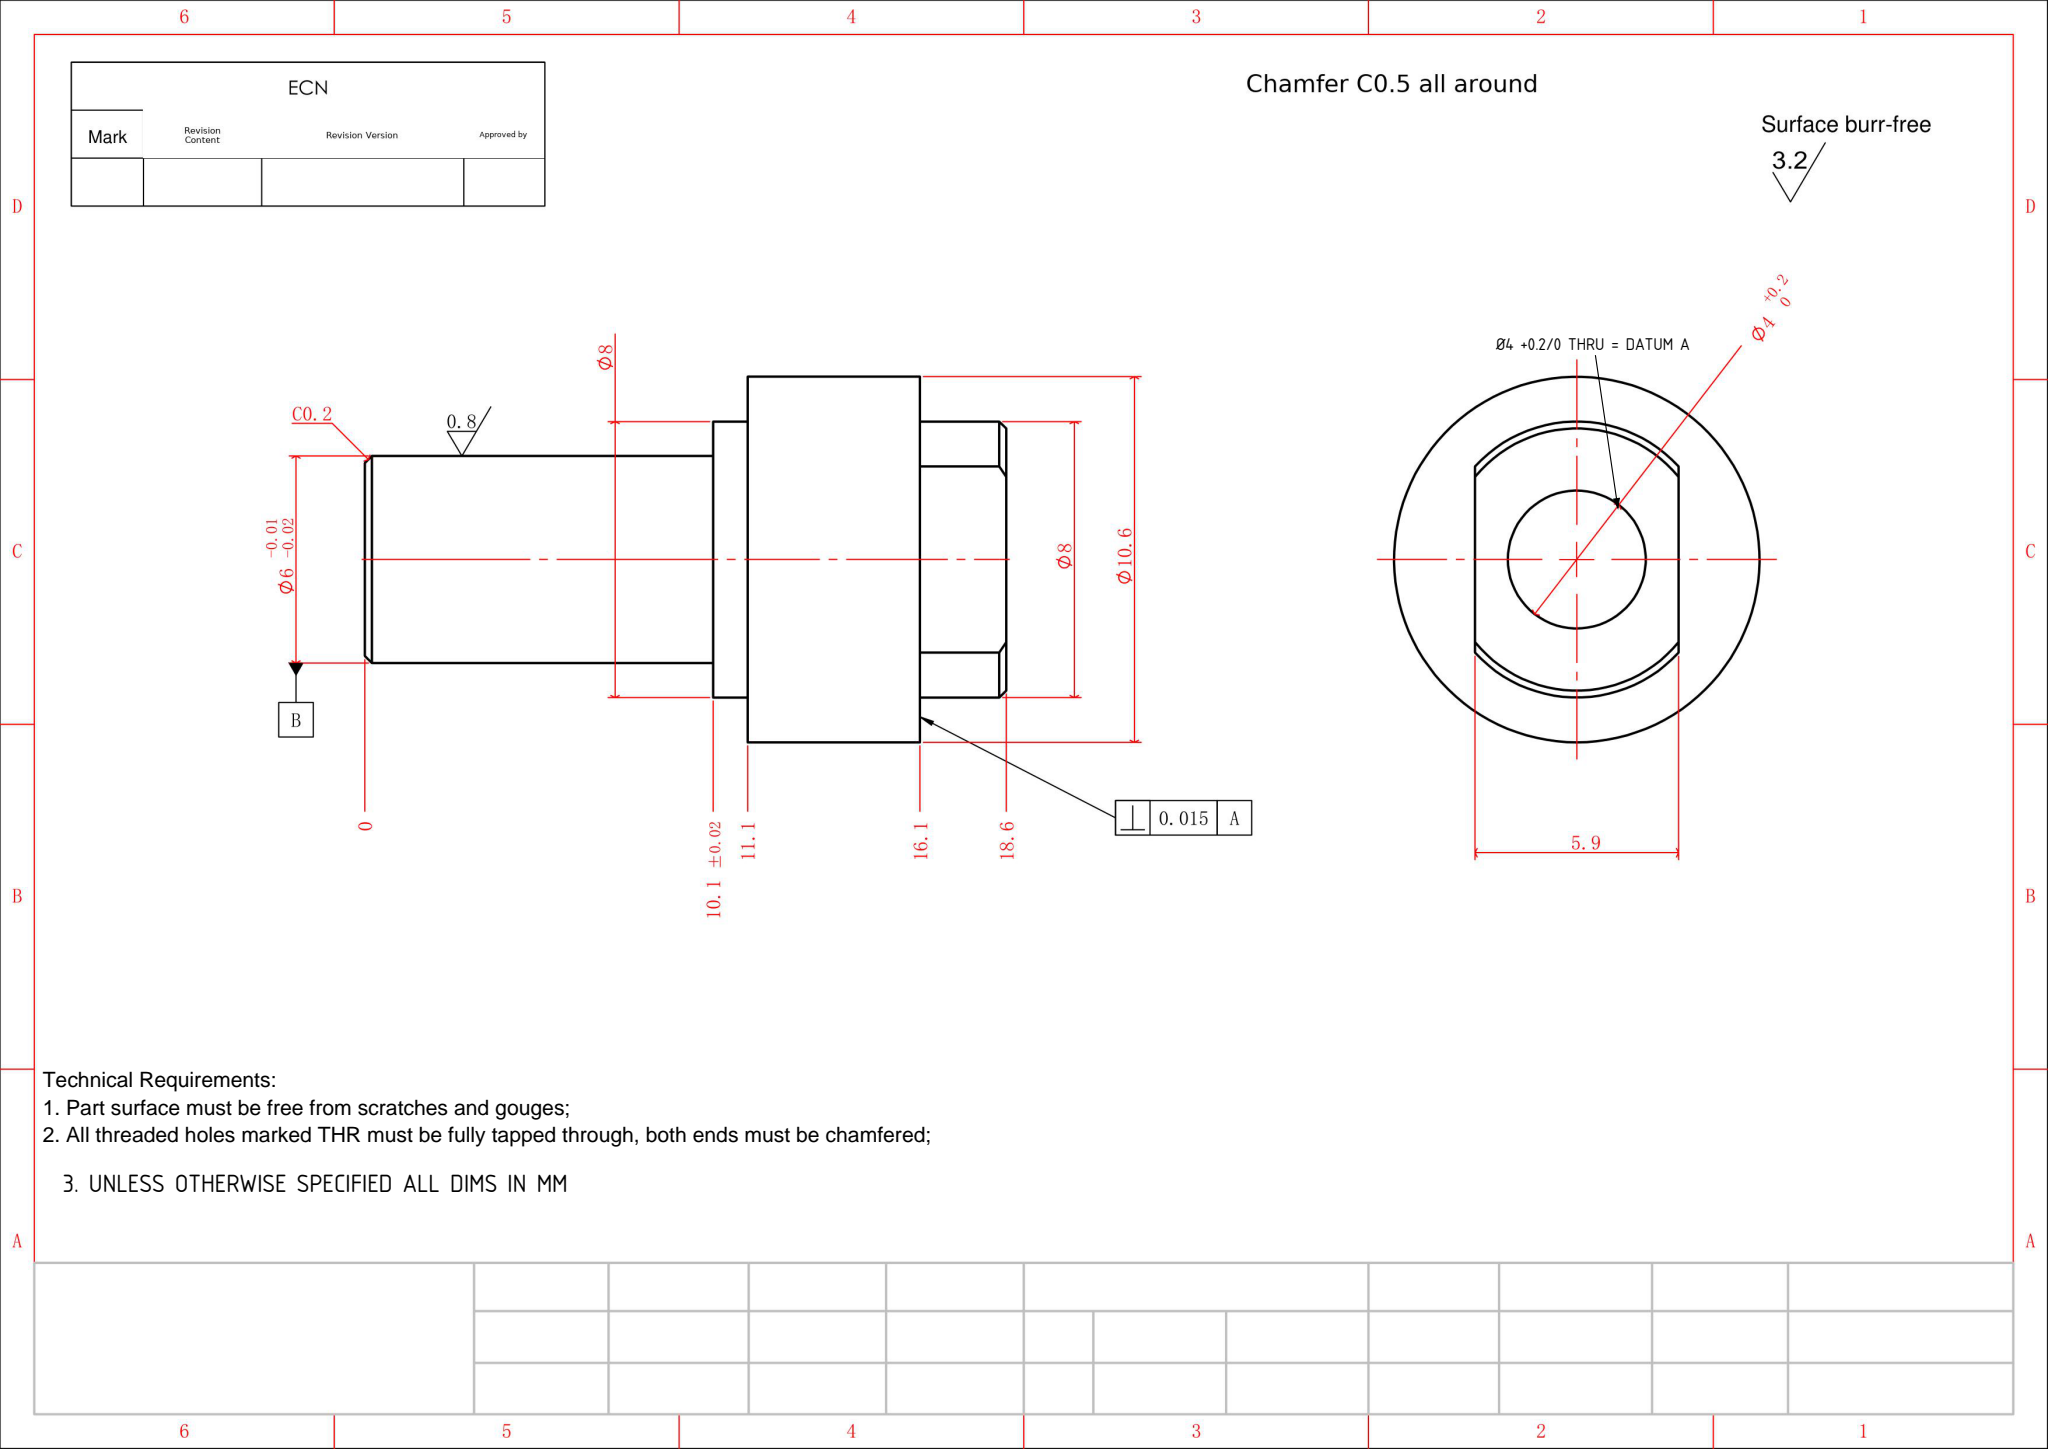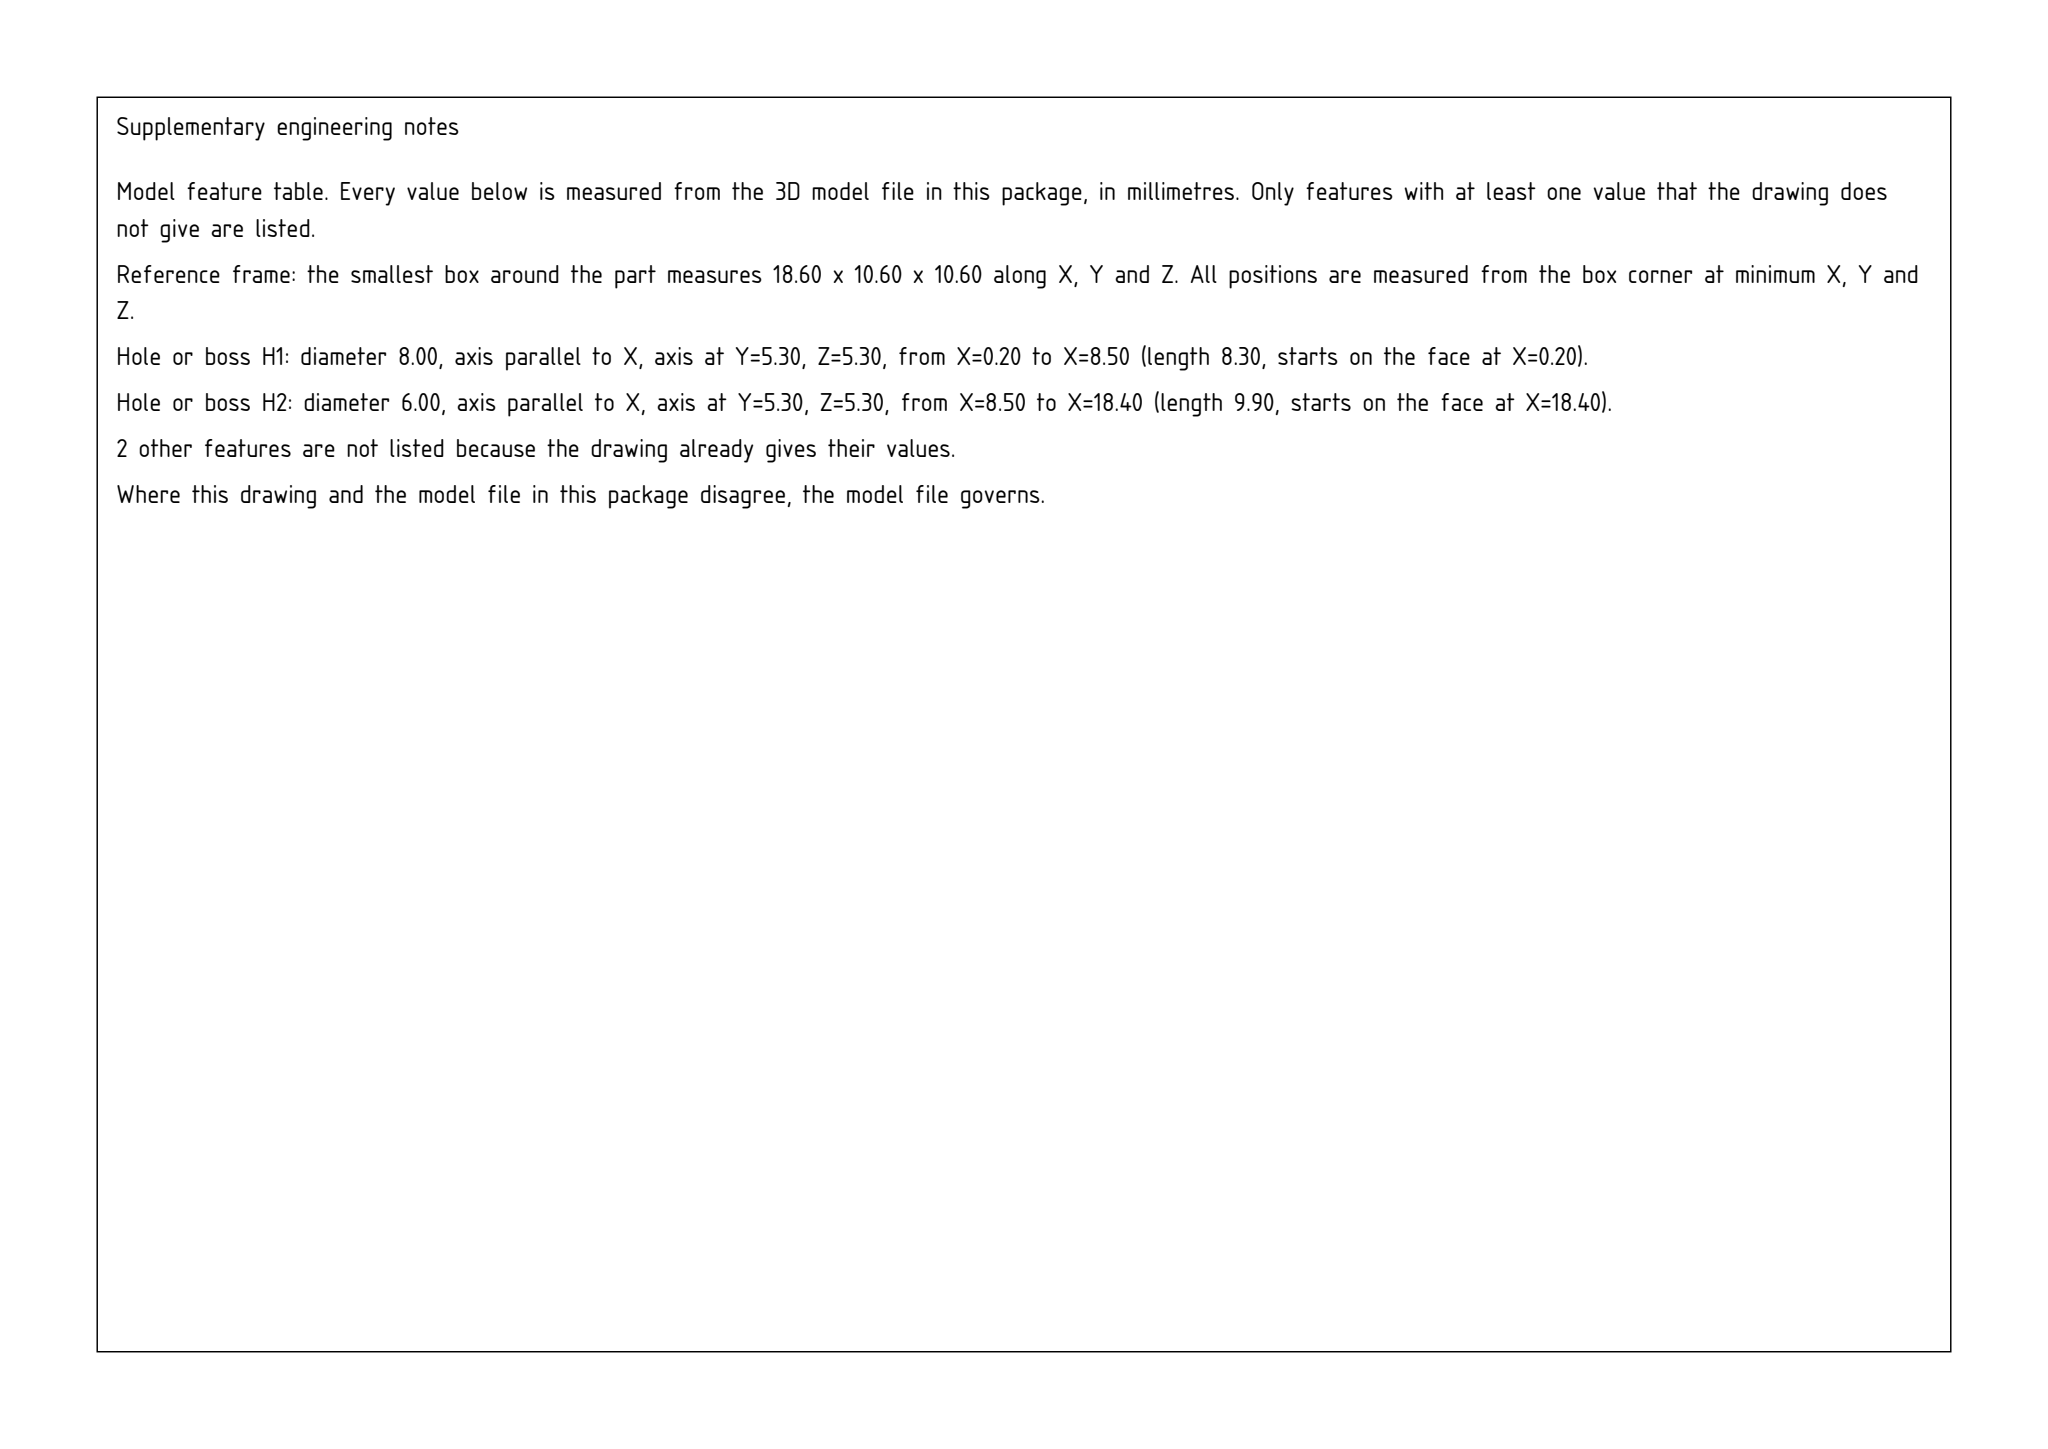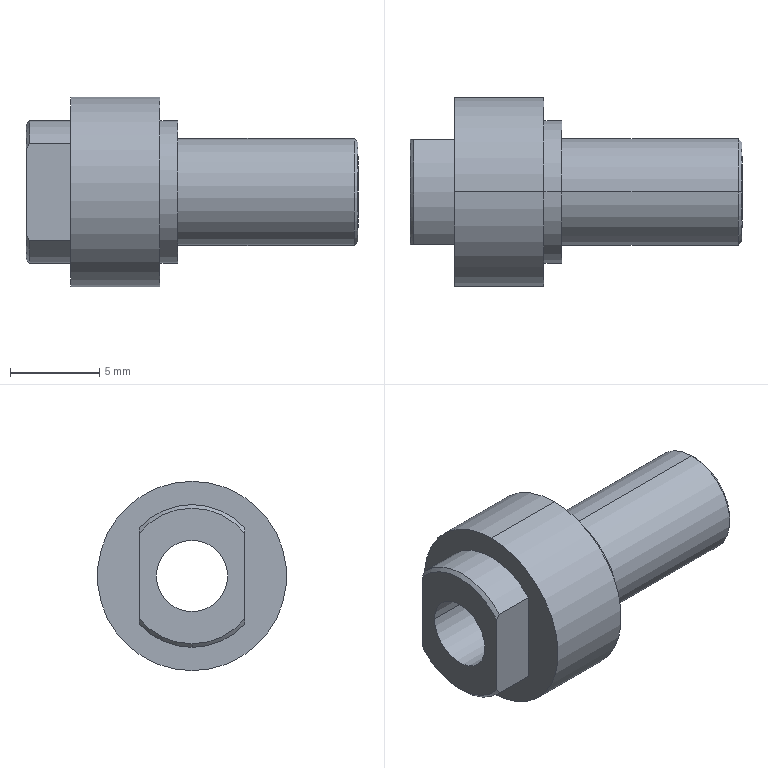Part | SolidWorks | mm | 1 solid | 23 faces | box 18.6 x 10.6 x 10.6 mm | volume 649 mm3 | cylinder 11 | plane 7 | cone 5 | commonest cylinder face diameters 8 x5 4 x2 6 x2 10.6 x2
Drawing notes:
DATUM A = AXIS OF Ø4 +0.2/0 THRU BORE | from the solid: Ø4.0 cylinder, axis x, centered at y=5.3 z=5.3, length 18.6 (full part)
UNLESS OTHERWISE SPECIFIED ALL DIMS IN MM | from the solid: STEP model units mm; bbox 18.6 x 10.6 x 10.6
STEP:
#1=CARTESIAN_POINT('',(-0.,-2.,0.));
#2=VERTEX_POINT('',#1);
#3=CARTESIAN_POINT('',(-0.,2.,0.));
#4=VERTEX_POINT('',#3);
#5=CARTESIAN_POINT('',(-0.,-0.,0.));
#6=DIRECTION('',(1.,0.,0.));
#7=DIRECTION('',(0.,1.,0.));
#8=AXIS2_PLACEMENT_3D('',#5,#6,#7);
#9=CIRCLE('',#8,2.);
#10=EDGE_CURVE('',#2,#4,#9,.T.);
#11=ORIENTED_EDGE('',*,*,#10,.F.);
#12=CARTESIAN_POINT('',(18.6,-2.,0.));
#13=VERTEX_POINT('',#12);
#14=CARTESIAN_POINT('',(-5.289,-2.,0.));
#15=DIRECTION('',(1.,0.,0.));
#16=VECTOR('',#15,1000.);
#17=LINE('',#14,#16);
#18=EDGE_CURVE('',#2,#13,#17,.T.);
#19=ORIENTED_EDGE('',*,*,#18,.T.);
#20=CARTESIAN_POINT('',(18.6,2.,0.));
#21=VERTEX_POINT('',#20);
#22=CARTESIAN_POINT('',(18.6,0.,0.));
#23=DIRECTION('',(-1.,-0.,0.));
#24=DIRECTION('',(0.,1.,0.));
#25=AXIS2_PLACEMENT_3D('',#22,#23,#24);
#26=CIRCLE('',#25,2.);
#27=EDGE_CURVE('',#21,#13,#26,.T.);
#28=ORIENTED_EDGE('',*,*,#27,.F.);
#29=CARTESIAN_POINT('',(-5.289,2.,0.));
#30=DIRECTION('',(1.,0.,0.));
#31=VECTOR('',#30,1000.);
#32=LINE('',#29,#31);
#33=EDGE_CURVE('',#4,#21,#32,.T.);
#34=ORIENTED_EDGE('',*,*,#33,.F.);
#35=EDGE_LOOP('',(#11,#19,#28,#34));
#36=FACE_OUTER_BOUND('',#35,.T.);
#37=CARTESIAN_POINT('',(-5.289,-0.,0.));
#38=DIRECTION('',(1.,0.,0.));
#39=DIRECTION('',(0.,1.,0.));
#40=AXIS2_PLACEMENT_3D('',#37,#38,#39);
#41=CYLINDRICAL_SURFACE('',#40,2.);
#42=ADVANCED_FACE('',(#36),#41,.F.);
#43=CARTESIAN_POINT('',(0.,0.,-3.8));
#44=VERTEX_POINT('',#43);
#45=CARTESIAN_POINT('',(-0.,-2.95,-2.395));
#46=VERTEX_POINT('',#45);
#47=CARTESIAN_POINT('',(0.,0.,0.));
#48=DIRECTION('',(-1.,0.,0.));
#49=DIRECTION('',(0.,0.,-1.));
#50=AXIS2_PLACEMENT_3D('',#47,#48,#49);
#51=CIRCLE('',#50,3.8);
#52=EDGE_CURVE('',#44,#46,#51,.T.);
#53=ORIENTED_EDGE('',*,*,#52,.F.);
#54=CARTESIAN_POINT('',(0.2,0.,-4.));
#55=VERTEX_POINT('',#54);
#56=CARTESIAN_POINT('',(0.2,0.,-4.));
#57=DIRECTION('',(0.7071,0.,-0.7071));
#58=VECTOR('',#57,1000.);
#59=LINE('',#56,#58);
#60=EDGE_CURVE('',#44,#55,#59,.T.);
#61=ORIENTED_EDGE('',*,*,#60,.T.);
#62=CARTESIAN_POINT('',(0.2,-2.95,-2.701));
#63=VERTEX_POINT('',#62);
#64=CARTESIAN_POINT('',(0.2,0.,0.));
#65=DIRECTION('',(-1.,-0.,0.));
#66=DIRECTION('',(-0.,1.,0.));
#67=AXIS2_PLACEMENT_3D('',#64,#65,#66);
#68=CIRCLE('',#67,4.);
#69=EDGE_CURVE('',#55,#63,#68,.T.);
#70=ORIENTED_EDGE('',*,*,#69,.T.);
#71=CARTESIAN_POINT('',(0.2,-2.95,-2.701));
#72=CARTESIAN_POINT('',(0.1318,-2.95,-2.6));
#73=CARTESIAN_POINT('',(0.06499,-2.95,-2.498));
#74=CARTESIAN_POINT('',(-0.,-2.95,-2.395));
#75=B_SPLINE_CURVE_WITH_KNOTS('',3,(#71,#72,#73,#74),.UNSPECIFIED.,.F.,.F.,(4,4),(0.,0.0003656),.UNSPECIFIED.);
#76=EDGE_CURVE('',#63,#46,#75,.T.);
#77=ORIENTED_EDGE('',*,*,#76,.T.);
#78=EDGE_LOOP('',(#53,#61,#70,#77));
#79=FACE_OUTER_BOUND('',#78,.T.);
#80=CARTESIAN_POINT('',(0.2,0.,0.));
#81=DIRECTION('',(1.,0.,0.));
#82=DIRECTION('',(0.,0.,-1.));
#83=AXIS2_PLACEMENT_3D('',#80,#81,#82);
#84=CONICAL_SURFACE('',#83,4.,0.7854);
#85=ADVANCED_FACE('',(#79),#84,.T.);
#86=CARTESIAN_POINT('',(18.6,0.,-2.8));
#87=VERTEX_POINT('',#86);
#88=CARTESIAN_POINT('',(18.6,0.,2.8));
#89=VERTEX_POINT('',#88);
#90=CARTESIAN_POINT('',(18.6,0.,0.));
#91=DIRECTION('',(1.,0.,0.));
#92=DIRECTION('',(0.,0.,1.));
#93=AXIS2_PLACEMENT_3D('',#90,#91,#92);
#94=CIRCLE('',#93,2.8);
#95=EDGE_CURVE('',#87,#89,#94,.T.);
#96=ORIENTED_EDGE('',*,*,#95,.F.);
#97=CARTESIAN_POINT('',(18.4,0.,-3.));
#98=VERTEX_POINT('',#97);
#99=CARTESIAN_POINT('',(18.4,0.,-3.));
#100=DIRECTION('',(-0.7071,0.,-0.7071));
#101=VECTOR('',#100,1000.);
#102=LINE('',#99,#101);
#103=EDGE_CURVE('',#87,#98,#102,.T.);
#104=ORIENTED_EDGE('',*,*,#103,.T.);
#105=CARTESIAN_POINT('',(18.4,0.,3.));
#106=VERTEX_POINT('',#105);
#107=CARTESIAN_POINT('',(18.4,0.,0.));
#108=DIRECTION('',(1.,0.,0.));
#109=DIRECTION('',(0.,-1.,0.));
#110=AXIS2_PLACEMENT_3D('',#107,#108,#109);
#111=CIRCLE('',#110,3.);
#112=EDGE_CURVE('',#98,#106,#111,.T.);
#113=ORIENTED_EDGE('',*,*,#112,.T.);
#114=CARTESIAN_POINT('',(18.4,0.,3.));
#115=DIRECTION('',(-0.7071,0.,0.7071));
#116=VECTOR('',#115,1000.);
#117=LINE('',#114,#116);
#118=EDGE_CURVE('',#89,#106,#117,.T.);
#119=ORIENTED_EDGE('',*,*,#118,.F.);
#120=EDGE_LOOP('',(#96,#104,#113,#119));
#121=FACE_OUTER_BOUND('',#120,.T.);
#122=CARTESIAN_POINT('',(18.4,0.,0.));
#123=DIRECTION('',(-1.,0.,0.));
#124=DIRECTION('',(0.,0.,1.));
#125=AXIS2_PLACEMENT_3D('',#122,#123,#124);
#126=CONICAL_SURFACE('',#125,3.,0.7854);
#127=ADVANCED_FACE('',(#121),#126,.T.);
#128=ORIENTED_EDGE('',*,*,#69,.F.);
#129=CARTESIAN_POINT('',(2.5,0.,-4.));
#130=VERTEX_POINT('',#129);
#131=CARTESIAN_POINT('',(1.25,0.,-4.));
#132=DIRECTION('',(1.,0.,0.));
#133=VECTOR('',#132,1000.);
#134=LINE('',#131,#133);
#135=EDGE_CURVE('',#55,#130,#134,.T.);
#136=ORIENTED_EDGE('',*,*,#135,.T.);
#137=CARTESIAN_POINT('',(2.5,-2.95,-2.701));
#138=VERTEX_POINT('',#137);
#139=CARTESIAN_POINT('',(2.5,0.,0.));
#140=DIRECTION('',(-1.,0.,0.));
#141=DIRECTION('',(0.,0.,-1.));
#142=AXIS2_PLACEMENT_3D('',#139,#140,#141);
#143=CIRCLE('',#142,4.);
#144=EDGE_CURVE('',#130,#138,#143,.T.);
#145=ORIENTED_EDGE('',*,*,#144,.T.);
#146=CARTESIAN_POINT('',(-0.,-2.95,-2.701));
#147=DIRECTION('',(-1.,0.,0.));
#148=VECTOR('',#147,1000.);
#149=LINE('',#146,#148);
#150=EDGE_CURVE('',#138,#63,#149,.T.);
#151=ORIENTED_EDGE('',*,*,#150,.T.);
#152=EDGE_LOOP('',(#128,#136,#145,#151));
#153=FACE_OUTER_BOUND('',#152,.T.);
#154=CARTESIAN_POINT('',(1.25,0.,0.));
#155=DIRECTION('',(1.,0.,0.));
#156=DIRECTION('',(0.,0.,-1.));
#157=AXIS2_PLACEMENT_3D('',#154,#155,#156);
#158=CYLINDRICAL_SURFACE('',#157,4.);
#159=ADVANCED_FACE('',(#153),#158,.T.);
#160=CARTESIAN_POINT('',(8.5,0.,-3.));
#161=VERTEX_POINT('',#160);
#162=CARTESIAN_POINT('',(8.5,0.,3.));
#163=VERTEX_POINT('',#162);
#164=CARTESIAN_POINT('',(8.5,0.,0.));
#165=DIRECTION('',(1.,0.,0.));
#166=DIRECTION('',(0.,0.,-1.));
#167=AXIS2_PLACEMENT_3D('',#164,#165,#166);
#168=CIRCLE('',#167,3.);
#169=EDGE_CURVE('',#161,#163,#168,.T.);
#170=ORIENTED_EDGE('',*,*,#169,.T.);
#171=CARTESIAN_POINT('',(13.55,0.,3.));
#172=DIRECTION('',(1.,0.,0.));
#173=VECTOR('',#172,1000.);
#174=LINE('',#171,#173);
#175=EDGE_CURVE('',#163,#106,#174,.T.);
#176=ORIENTED_EDGE('',*,*,#175,.T.);
#177=ORIENTED_EDGE('',*,*,#112,.F.);
#178=CARTESIAN_POINT('',(13.55,0.,-3.));
#179=DIRECTION('',(1.,0.,0.));
#180=VECTOR('',#179,1000.);
#181=LINE('',#178,#180);
#182=EDGE_CURVE('',#161,#98,#181,.T.);
#183=ORIENTED_EDGE('',*,*,#182,.F.);
#184=EDGE_LOOP('',(#170,#176,#177,#183));
#185=FACE_OUTER_BOUND('',#184,.T.);
#186=CARTESIAN_POINT('',(13.55,0.,0.));
#187=DIRECTION('',(1.,0.,0.));
#188=DIRECTION('',(0.,0.,-1.));
#189=AXIS2_PLACEMENT_3D('',#186,#187,#188);
#190=CYLINDRICAL_SURFACE('',#189,3.);
#191=ADVANCED_FACE('',(#185),#190,.T.);
#192=CARTESIAN_POINT('',(2.5,0.,5.3));
#193=VERTEX_POINT('',#192);
#194=CARTESIAN_POINT('',(2.5,0.,-5.3));
#195=VERTEX_POINT('',#194);
#196=CARTESIAN_POINT('',(2.5,0.,0.));
#197=DIRECTION('',(-1.,0.,0.));
#198=DIRECTION('',(0.,0.,-1.));
#199=AXIS2_PLACEMENT_3D('',#196,#197,#198);
#200=CIRCLE('',#199,5.3);
#201=EDGE_CURVE('',#193,#195,#200,.T.);
#202=ORIENTED_EDGE('',*,*,#201,.F.);
#203=CARTESIAN_POINT('',(7.5,0.,5.3));
#204=VERTEX_POINT('',#203);
#205=CARTESIAN_POINT('',(5.5,0.,5.3));
#206=DIRECTION('',(1.,0.,0.));
#207=VECTOR('',#206,1000.);
#208=LINE('',#205,#207);
#209=EDGE_CURVE('',#193,#204,#208,.T.);
#210=ORIENTED_EDGE('',*,*,#209,.T.);
#211=CARTESIAN_POINT('',(7.5,0.,-5.3));
#212=VERTEX_POINT('',#211);
#213=CARTESIAN_POINT('',(7.5,0.,0.));
#214=DIRECTION('',(-1.,0.,0.));
#215=DIRECTION('',(0.,0.,-1.));
#216=AXIS2_PLACEMENT_3D('',#213,#214,#215);
#217=CIRCLE('',#216,5.3);
#218=EDGE_CURVE('',#204,#212,#217,.T.);
#219=ORIENTED_EDGE('',*,*,#218,.T.);
#220=CARTESIAN_POINT('',(5.5,0.,-5.3));
#221=DIRECTION('',(1.,0.,0.));
#222=VECTOR('',#221,1000.);
#223=LINE('',#220,#222);
#224=EDGE_CURVE('',#195,#212,#223,.T.);
#225=ORIENTED_EDGE('',*,*,#224,.F.);
#226=EDGE_LOOP('',(#202,#210,#219,#225));
#227=FACE_OUTER_BOUND('',#226,.T.);
#228=CARTESIAN_POINT('',(5.5,0.,0.));
#229=DIRECTION('',(1.,0.,0.));
#230=DIRECTION('',(0.,0.,-1.));
#231=AXIS2_PLACEMENT_3D('',#228,#229,#230);
#232=CYLINDRICAL_SURFACE('',#231,5.3);
#233=ADVANCED_FACE('',(#227),#232,.T.);
#234=CARTESIAN_POINT('',(7.5,0.,-4.));
#235=VERTEX_POINT('',#234);
#236=CARTESIAN_POINT('',(7.5,0.,4.));
#237=VERTEX_POINT('',#236);
#238=CARTESIAN_POINT('',(7.5,0.,0.));
#239=DIRECTION('',(1.,0.,0.));
#240=DIRECTION('',(0.,0.,-1.));
#241=AXIS2_PLACEMENT_3D('',#238,#239,#240);
#242=CIRCLE('',#241,4.);
#243=EDGE_CURVE('',#235,#237,#242,.T.);
#244=ORIENTED_EDGE('',*,*,#243,.T.);
#245=CARTESIAN_POINT('',(8.5,0.,4.));
#246=VERTEX_POINT('',#245);
#247=CARTESIAN_POINT('',(8.,0.,4.));
#248=DIRECTION('',(1.,0.,0.));
#249=VECTOR('',#248,1000.);
#250=LINE('',#247,#249);
#251=EDGE_CURVE('',#237,#246,#250,.T.);
#252=ORIENTED_EDGE('',*,*,#251,.T.);
#253=CARTESIAN_POINT('',(8.5,0.,-4.));
#254=VERTEX_POINT('',#253);
#255=CARTESIAN_POINT('',(8.5,0.,0.));
#256=DIRECTION('',(1.,0.,0.));
#257=DIRECTION('',(0.,0.,-1.));
#258=AXIS2_PLACEMENT_3D('',#255,#256,#257);
#259=CIRCLE('',#258,4.);
#260=EDGE_CURVE('',#254,#246,#259,.T.);
#261=ORIENTED_EDGE('',*,*,#260,.F.);
#262=CARTESIAN_POINT('',(8.,0.,-4.));
#263=DIRECTION('',(1.,0.,0.));
#264=VECTOR('',#263,1000.);
#265=LINE('',#262,#264);
#266=EDGE_CURVE('',#235,#254,#265,.T.);
#267=ORIENTED_EDGE('',*,*,#266,.F.);
#268=EDGE_LOOP('',(#244,#252,#261,#267));
#269=FACE_OUTER_BOUND('',#268,.T.);
#270=CARTESIAN_POINT('',(8.,0.,0.));
#271=DIRECTION('',(1.,0.,0.));
#272=DIRECTION('',(0.,0.,-1.));
#273=AXIS2_PLACEMENT_3D('',#270,#271,#272);
#274=CYLINDRICAL_SURFACE('',#273,4.);
#275=ADVANCED_FACE('',(#269),#274,.T.);
#276=ORIENTED_EDGE('',*,*,#18,.F.);
#277=CARTESIAN_POINT('',(-0.,-0.,0.));
#278=DIRECTION('',(1.,0.,0.));
#279=DIRECTION('',(0.,1.,0.));
#280=AXIS2_PLACEMENT_3D('',#277,#278,#279);
#281=CIRCLE('',#280,2.);
#282=EDGE_CURVE('',#4,#2,#281,.T.);
#283=ORIENTED_EDGE('',*,*,#282,.F.);
#284=ORIENTED_EDGE('',*,*,#33,.T.);
#285=CARTESIAN_POINT('',(18.6,0.,0.));
#286=DIRECTION('',(-1.,-0.,0.));
#287=DIRECTION('',(0.,1.,0.));
#288=AXIS2_PLACEMENT_3D('',#285,#286,#287);
#289=CIRCLE('',#288,2.);
#290=EDGE_CURVE('',#13,#21,#289,.T.);
#291=ORIENTED_EDGE('',*,*,#290,.F.);
#292=EDGE_LOOP('',(#276,#283,#284,#291));
#293=FACE_OUTER_BOUND('',#292,.T.);
#294=CARTESIAN_POINT('',(-5.289,-0.,0.));
#295=DIRECTION('',(1.,0.,0.));
#296=DIRECTION('',(0.,1.,0.));
#297=AXIS2_PLACEMENT_3D('',#294,#295,#296);
#298=CYLINDRICAL_SURFACE('',#297,2.);
#299=ADVANCED_FACE('',(#293),#298,.F.);
#300=ORIENTED_EDGE('',*,*,#282,.T.);
#301=ORIENTED_EDGE('',*,*,#10,.T.);
#302=EDGE_LOOP('',(#300,#301));
#303=FACE_BOUND('',#302,.T.);
#304=CARTESIAN_POINT('',(-0.,2.95,-2.395));
#305=VERTEX_POINT('',#304);
#306=CARTESIAN_POINT('',(0.,0.,0.));
#307=DIRECTION('',(-1.,0.,0.));
#308=DIRECTION('',(0.,0.,-1.));
#309=AXIS2_PLACEMENT_3D('',#306,#307,#308);
#310=CIRCLE('',#309,3.8);
#311=EDGE_CURVE('',#305,#44,#310,.T.);
#312=ORIENTED_EDGE('',*,*,#311,.T.);
#313=ORIENTED_EDGE('',*,*,#52,.T.);
#314=CARTESIAN_POINT('',(-0.,-2.95,2.395));
#315=VERTEX_POINT('',#314);
#316=CARTESIAN_POINT('',(-0.,-2.95,0.));
#317=DIRECTION('',(0.,0.,1.));
#318=VECTOR('',#317,1000.);
#319=LINE('',#316,#318);
#320=EDGE_CURVE('',#46,#315,#319,.T.);
#321=ORIENTED_EDGE('',*,*,#320,.T.);
#322=CARTESIAN_POINT('',(-0.,2.95,2.395));
#323=VERTEX_POINT('',#322);
#324=CARTESIAN_POINT('',(0.,0.,0.));
#325=DIRECTION('',(-1.,0.,0.));
#326=DIRECTION('',(0.,0.,-1.));
#327=AXIS2_PLACEMENT_3D('',#324,#325,#326);
#328=CIRCLE('',#327,3.8);
#329=EDGE_CURVE('',#315,#323,#328,.T.);
#330=ORIENTED_EDGE('',*,*,#329,.T.);
#331=CARTESIAN_POINT('',(-0.,2.95,0.));
#332=DIRECTION('',(0.,0.,-1.));
#333=VECTOR('',#332,1000.);
#334=LINE('',#331,#333);
#335=EDGE_CURVE('',#323,#305,#334,.T.);
#336=ORIENTED_EDGE('',*,*,#335,.T.);
#337=EDGE_LOOP('',(#312,#313,#321,#330,#336));
#338=FACE_OUTER_BOUND('',#337,.T.);
#339=CARTESIAN_POINT('',(-0.,2.,0.));
#340=DIRECTION('',(-1.,-0.,0.));
#341=DIRECTION('',(0.,-1.,0.));
#342=AXIS2_PLACEMENT_3D('',#339,#340,#341);
#343=PLANE('',#342);
#344=ADVANCED_FACE('',(#303,#338),#343,.T.);
#345=ORIENTED_EDGE('',*,*,#27,.T.);
#346=ORIENTED_EDGE('',*,*,#290,.T.);
#347=EDGE_LOOP('',(#345,#346));
#348=FACE_BOUND('',#347,.T.);
#349=CARTESIAN_POINT('',(18.6,0.,0.));
#350=DIRECTION('',(1.,0.,0.));
#351=DIRECTION('',(0.,0.,1.));
#352=AXIS2_PLACEMENT_3D('',#349,#350,#351);
#353=CIRCLE('',#352,2.8);
#354=EDGE_CURVE('',#89,#87,#353,.T.);
#355=ORIENTED_EDGE('',*,*,#354,.T.);
#356=ORIENTED_EDGE('',*,*,#95,.T.);
#357=EDGE_LOOP('',(#355,#356));
#358=FACE_OUTER_BOUND('',#357,.T.);
#359=CARTESIAN_POINT('',(18.6,1.5,0.));
#360=DIRECTION('',(1.,0.,0.));
#361=DIRECTION('',(0.,0.,-1.));
#362=AXIS2_PLACEMENT_3D('',#359,#360,#361);
#363=PLANE('',#362);
#364=ADVANCED_FACE('',(#348,#358),#363,.T.);
#365=ORIENTED_EDGE('',*,*,#320,.F.);
#366=ORIENTED_EDGE('',*,*,#76,.F.);
#367=ORIENTED_EDGE('',*,*,#150,.F.);
#368=CARTESIAN_POINT('',(2.5,-2.95,2.701));
#369=VERTEX_POINT('',#368);
#370=CARTESIAN_POINT('',(2.5,-2.95,2.701));
#371=DIRECTION('',(0.,0.,-1.));
#372=VECTOR('',#371,1000.);
#373=LINE('',#370,#372);
#374=EDGE_CURVE('',#369,#138,#373,.T.);
#375=ORIENTED_EDGE('',*,*,#374,.F.);
#376=CARTESIAN_POINT('',(0.2,-2.95,2.701));
#377=VERTEX_POINT('',#376);
#378=CARTESIAN_POINT('',(-0.,-2.95,2.701));
#379=DIRECTION('',(1.,0.,0.));
#380=VECTOR('',#379,1000.);
#381=LINE('',#378,#380);
#382=EDGE_CURVE('',#377,#369,#381,.T.);
#383=ORIENTED_EDGE('',*,*,#382,.F.);
#384=CARTESIAN_POINT('',(-0.,-2.95,2.395));
#385=CARTESIAN_POINT('',(0.06499,-2.95,2.498));
#386=CARTESIAN_POINT('',(0.1318,-2.95,2.6));
#387=CARTESIAN_POINT('',(0.2,-2.95,2.701));
#388=B_SPLINE_CURVE_WITH_KNOTS('',3,(#384,#385,#386,#387),.UNSPECIFIED.,.F.,.F.,(4,4),(0.,0.0003656),.UNSPECIFIED.);
#389=EDGE_CURVE('',#315,#377,#388,.T.);
#390=ORIENTED_EDGE('',*,*,#389,.F.);
#391=EDGE_LOOP('',(#365,#366,#367,#375,#383,#390));
#392=FACE_OUTER_BOUND('',#391,.T.);
#393=CARTESIAN_POINT('',(-0.,-2.95,2.701));
#394=DIRECTION('',(0.,1.,0.));
#395=DIRECTION('',(0.,0.,1.));
#396=AXIS2_PLACEMENT_3D('',#393,#394,#395);
#397=PLANE('',#396);
#398=ADVANCED_FACE('',(#392),#397,.F.);
#399=ORIENTED_EDGE('',*,*,#60,.F.);
#400=ORIENTED_EDGE('',*,*,#311,.F.);
#401=CARTESIAN_POINT('',(0.2,2.95,-2.701));
#402=VERTEX_POINT('',#401);
#403=CARTESIAN_POINT('',(-0.,2.95,-2.395));
#404=CARTESIAN_POINT('',(0.06499,2.95,-2.498));
#405=CARTESIAN_POINT('',(0.1318,2.95,-2.6));
#406=CARTESIAN_POINT('',(0.2,2.95,-2.701));
#407=B_SPLINE_CURVE_WITH_KNOTS('',3,(#403,#404,#405,#406),.UNSPECIFIED.,.F.,.F.,(4,4),(0.,0.0003656),.UNSPECIFIED.);
#408=EDGE_CURVE('',#305,#402,#407,.T.);
#409=ORIENTED_EDGE('',*,*,#408,.T.);
#410=CARTESIAN_POINT('',(0.2,0.,0.));
#411=DIRECTION('',(-1.,-0.,0.));
#412=DIRECTION('',(-0.,1.,0.));
#413=AXIS2_PLACEMENT_3D('',#410,#411,#412);
#414=CIRCLE('',#413,4.);
#415=EDGE_CURVE('',#402,#55,#414,.T.);
#416=ORIENTED_EDGE('',*,*,#415,.T.);
#417=EDGE_LOOP('',(#399,#400,#409,#416));
#418=FACE_OUTER_BOUND('',#417,.T.);
#419=CARTESIAN_POINT('',(0.2,0.,0.));
#420=DIRECTION('',(1.,0.,0.));
#421=DIRECTION('',(0.,0.,-1.));
#422=AXIS2_PLACEMENT_3D('',#419,#420,#421);
#423=CONICAL_SURFACE('',#422,4.,0.7854);
#424=ADVANCED_FACE('',(#418),#423,.T.);
#425=CARTESIAN_POINT('',(2.5,2.95,2.701));
#426=VERTEX_POINT('',#425);
#427=CARTESIAN_POINT('',(0.2,2.95,2.701));
#428=VERTEX_POINT('',#427);
#429=CARTESIAN_POINT('',(-0.,2.95,2.701));
#430=DIRECTION('',(-1.,0.,0.));
#431=VECTOR('',#430,1000.);
#432=LINE('',#429,#431);
#433=EDGE_CURVE('',#426,#428,#432,.T.);
#434=ORIENTED_EDGE('',*,*,#433,.F.);
#435=CARTESIAN_POINT('',(2.5,2.95,-2.701));
#436=VERTEX_POINT('',#435);
#437=CARTESIAN_POINT('',(2.5,2.95,-2.701));
#438=DIRECTION('',(0.,0.,1.));
#439=VECTOR('',#438,1000.);
#440=LINE('',#437,#439);
#441=EDGE_CURVE('',#436,#426,#440,.T.);
#442=ORIENTED_EDGE('',*,*,#441,.F.);
#443=CARTESIAN_POINT('',(-0.,2.95,-2.701));
#444=DIRECTION('',(1.,0.,0.));
#445=VECTOR('',#444,1000.);
#446=LINE('',#443,#445);
#447=EDGE_CURVE('',#402,#436,#446,.T.);
#448=ORIENTED_EDGE('',*,*,#447,.F.);
#449=ORIENTED_EDGE('',*,*,#408,.F.);
#450=ORIENTED_EDGE('',*,*,#335,.F.);
#451=CARTESIAN_POINT('',(0.2,2.95,2.701));
#452=CARTESIAN_POINT('',(0.1318,2.95,2.6));
#453=CARTESIAN_POINT('',(0.06499,2.95,2.498));
#454=CARTESIAN_POINT('',(-0.,2.95,2.395));
#455=B_SPLINE_CURVE_WITH_KNOTS('',3,(#451,#452,#453,#454),.UNSPECIFIED.,.F.,.F.,(4,4),(0.,0.0003656),.UNSPECIFIED.);
#456=EDGE_CURVE('',#428,#323,#455,.T.);
#457=ORIENTED_EDGE('',*,*,#456,.F.);
#458=EDGE_LOOP('',(#434,#442,#448,#449,#450,#457));
#459=FACE_OUTER_BOUND('',#458,.T.);
#460=CARTESIAN_POINT('',(-0.,2.95,-2.701));
#461=DIRECTION('',(0.,-1.,0.));
#462=DIRECTION('',(0.,0.,-1.));
#463=AXIS2_PLACEMENT_3D('',#460,#461,#462);
#464=PLANE('',#463);
#465=ADVANCED_FACE('',(#459),#464,.F.);
#466=ORIENTED_EDGE('',*,*,#456,.T.);
#467=ORIENTED_EDGE('',*,*,#329,.F.);
#468=ORIENTED_EDGE('',*,*,#389,.T.);
#469=CARTESIAN_POINT('',(0.2,0.,0.));
#470=DIRECTION('',(-1.,-0.,0.));
#471=DIRECTION('',(-0.,1.,0.));
#472=AXIS2_PLACEMENT_3D('',#469,#470,#471);
#473=CIRCLE('',#472,4.);
#474=EDGE_CURVE('',#377,#428,#473,.T.);
#475=ORIENTED_EDGE('',*,*,#474,.T.);
#476=EDGE_LOOP('',(#466,#467,#468,#475));
#477=FACE_OUTER_BOUND('',#476,.T.);
#478=CARTESIAN_POINT('',(0.2,0.,0.));
#479=DIRECTION('',(1.,0.,0.));
#480=DIRECTION('',(0.,0.,-1.));
#481=AXIS2_PLACEMENT_3D('',#478,#479,#480);
#482=CONICAL_SURFACE('',#481,4.,0.7854);
#483=ADVANCED_FACE('',(#477),#482,.T.);
#484=ORIENTED_EDGE('',*,*,#103,.F.);
#485=ORIENTED_EDGE('',*,*,#354,.F.);
#486=ORIENTED_EDGE('',*,*,#118,.T.);
#487=CARTESIAN_POINT('',(18.4,0.,0.));
#488=DIRECTION('',(1.,0.,0.));
#489=DIRECTION('',(0.,-1.,0.));
#490=AXIS2_PLACEMENT_3D('',#487,#488,#489);
#491=CIRCLE('',#490,3.);
#492=EDGE_CURVE('',#106,#98,#491,.T.);
#493=ORIENTED_EDGE('',*,*,#492,.T.);
#494=EDGE_LOOP('',(#484,#485,#486,#493));
#495=FACE_OUTER_BOUND('',#494,.T.);
#496=CARTESIAN_POINT('',(18.4,0.,0.));
#497=DIRECTION('',(-1.,0.,0.));
#498=DIRECTION('',(0.,0.,1.));
#499=AXIS2_PLACEMENT_3D('',#496,#497,#498);
#500=CONICAL_SURFACE('',#499,3.,0.7854);
#501=ADVANCED_FACE('',(#495),#500,.T.);
#502=ORIENTED_EDGE('',*,*,#135,.F.);
#503=ORIENTED_EDGE('',*,*,#415,.F.);
#504=ORIENTED_EDGE('',*,*,#447,.T.);
#505=CARTESIAN_POINT('',(2.5,0.,0.));
#506=DIRECTION('',(-1.,0.,0.));
#507=DIRECTION('',(0.,-0.,-1.));
#508=AXIS2_PLACEMENT_3D('',#505,#506,#507);
#509=CIRCLE('',#508,4.);
#510=EDGE_CURVE('',#436,#130,#509,.T.);
#511=ORIENTED_EDGE('',*,*,#510,.T.);
#512=EDGE_LOOP('',(#502,#503,#504,#511));
#513=FACE_OUTER_BOUND('',#512,.T.);
#514=CARTESIAN_POINT('',(1.25,0.,0.));
#515=DIRECTION('',(1.,0.,0.));
#516=DIRECTION('',(0.,0.,-1.));
#517=AXIS2_PLACEMENT_3D('',#514,#515,#516);
#518=CYLINDRICAL_SURFACE('',#517,4.);
#519=ADVANCED_FACE('',(#513),#518,.T.);
#520=ORIENTED_EDGE('',*,*,#510,.F.);
#521=ORIENTED_EDGE('',*,*,#441,.T.);
#522=CARTESIAN_POINT('',(2.5,0.,0.));
#523=DIRECTION('',(1.,0.,0.));
#524=DIRECTION('',(0.,0.,-1.));
#525=AXIS2_PLACEMENT_3D('',#522,#523,#524);
#526=CIRCLE('',#525,4.);
#527=EDGE_CURVE('',#426,#369,#526,.T.);
#528=ORIENTED_EDGE('',*,*,#527,.T.);
#529=ORIENTED_EDGE('',*,*,#374,.T.);
#530=ORIENTED_EDGE('',*,*,#144,.F.);
#531=EDGE_LOOP('',(#520,#521,#528,#529,#530));
#532=FACE_BOUND('',#531,.T.);
#533=CARTESIAN_POINT('',(2.5,0.,0.));
#534=DIRECTION('',(-1.,0.,0.));
#535=DIRECTION('',(0.,0.,-1.));
#536=AXIS2_PLACEMENT_3D('',#533,#534,#535);
#537=CIRCLE('',#536,5.3);
#538=EDGE_CURVE('',#195,#193,#537,.T.);
#539=ORIENTED_EDGE('',*,*,#538,.T.);
#540=ORIENTED_EDGE('',*,*,#201,.T.);
#541=EDGE_LOOP('',(#539,#540));
#542=FACE_OUTER_BOUND('',#541,.T.);
#543=CARTESIAN_POINT('',(2.5,2.65,0.));
#544=DIRECTION('',(-1.,-0.,0.));
#545=DIRECTION('',(0.,-1.,0.));
#546=AXIS2_PLACEMENT_3D('',#543,#544,#545);
#547=PLANE('',#546);
#548=ADVANCED_FACE('',(#532,#542),#547,.T.);
#549=ORIENTED_EDGE('',*,*,#527,.F.);
#550=ORIENTED_EDGE('',*,*,#433,.T.);
#551=ORIENTED_EDGE('',*,*,#474,.F.);
#552=ORIENTED_EDGE('',*,*,#382,.T.);
#553=EDGE_LOOP('',(#549,#550,#551,#552));
#554=FACE_OUTER_BOUND('',#553,.T.);
#555=CARTESIAN_POINT('',(1.25,0.,0.));
#556=DIRECTION('',(1.,0.,0.));
#557=DIRECTION('',(0.,0.,-1.));
#558=AXIS2_PLACEMENT_3D('',#555,#556,#557);
#559=CYLINDRICAL_SURFACE('',#558,4.);
#560=ADVANCED_FACE('',(#554),#559,.T.);
#561=ORIENTED_EDGE('',*,*,#175,.F.);
#562=CARTESIAN_POINT('',(8.5,0.,0.));
#563=DIRECTION('',(1.,0.,0.));
#564=DIRECTION('',(0.,0.,-1.));
#565=AXIS2_PLACEMENT_3D('',#562,#563,#564);
#566=CIRCLE('',#565,3.);
#567=EDGE_CURVE('',#163,#161,#566,.T.);
#568=ORIENTED_EDGE('',*,*,#567,.T.);
#569=ORIENTED_EDGE('',*,*,#182,.T.);
#570=ORIENTED_EDGE('',*,*,#492,.F.);
#571=EDGE_LOOP('',(#561,#568,#569,#570));
#572=FACE_OUTER_BOUND('',#571,.T.);
#573=CARTESIAN_POINT('',(13.55,0.,0.));
#574=DIRECTION('',(1.,0.,0.));
#575=DIRECTION('',(0.,0.,-1.));
#576=AXIS2_PLACEMENT_3D('',#573,#574,#575);
#577=CYLINDRICAL_SURFACE('',#576,3.);
#578=ADVANCED_FACE('',(#572),#577,.T.);
#579=ORIENTED_EDGE('',*,*,#209,.F.);
#580=ORIENTED_EDGE('',*,*,#538,.F.);
#581=ORIENTED_EDGE('',*,*,#224,.T.);
#582=CARTESIAN_POINT('',(7.5,0.,0.));
#583=DIRECTION('',(-1.,0.,0.));
#584=DIRECTION('',(0.,0.,-1.));
#585=AXIS2_PLACEMENT_3D('',#582,#583,#584);
#586=CIRCLE('',#585,5.3);
#587=EDGE_CURVE('',#212,#204,#586,.T.);
#588=ORIENTED_EDGE('',*,*,#587,.T.);
#589=EDGE_LOOP('',(#579,#580,#581,#588));
#590=FACE_OUTER_BOUND('',#589,.T.);
#591=CARTESIAN_POINT('',(5.5,0.,0.));
#592=DIRECTION('',(1.,0.,0.));
#593=DIRECTION('',(0.,0.,-1.));
#594=AXIS2_PLACEMENT_3D('',#591,#592,#593);
#595=CYLINDRICAL_SURFACE('',#594,5.3);
#596=ADVANCED_FACE('',(#590),#595,.T.);
#597=ORIENTED_EDGE('',*,*,#169,.F.);
#598=ORIENTED_EDGE('',*,*,#567,.F.);
#599=EDGE_LOOP('',(#597,#598));
#600=FACE_BOUND('',#599,.T.);
#601=ORIENTED_EDGE('',*,*,#260,.T.);
#602=CARTESIAN_POINT('',(8.5,0.,0.));
#603=DIRECTION('',(1.,0.,0.));
#604=DIRECTION('',(0.,0.,-1.));
#605=AXIS2_PLACEMENT_3D('',#602,#603,#604);
#606=CIRCLE('',#605,4.);
#607=EDGE_CURVE('',#246,#254,#606,.T.);
#608=ORIENTED_EDGE('',*,*,#607,.T.);
#609=EDGE_LOOP('',(#601,#608));
#610=FACE_OUTER_BOUND('',#609,.T.);
#611=CARTESIAN_POINT('',(8.5,2.65,0.));
#612=DIRECTION('',(1.,0.,0.));
#613=DIRECTION('',(0.,0.,-1.));
#614=AXIS2_PLACEMENT_3D('',#611,#612,#613);
#615=PLANE('',#614);
#616=ADVANCED_FACE('',(#600,#610),#615,.T.);
#617=ORIENTED_EDGE('',*,*,#243,.F.);
#618=CARTESIAN_POINT('',(7.5,0.,0.));
#619=DIRECTION('',(1.,0.,0.));
#620=DIRECTION('',(0.,0.,-1.));
#621=AXIS2_PLACEMENT_3D('',#618,#619,#620);
#622=CIRCLE('',#621,4.);
#623=EDGE_CURVE('',#237,#235,#622,.T.);
#624=ORIENTED_EDGE('',*,*,#623,.F.);
#625=EDGE_LOOP('',(#617,#624));
#626=FACE_BOUND('',#625,.T.);
#627=ORIENTED_EDGE('',*,*,#587,.F.);
#628=ORIENTED_EDGE('',*,*,#218,.F.);
#629=EDGE_LOOP('',(#627,#628));
#630=FACE_OUTER_BOUND('',#629,.T.);
#631=CARTESIAN_POINT('',(7.5,4.65,0.));
#632=DIRECTION('',(-1.,-0.,0.));
#633=DIRECTION('',(0.,-1.,0.));
#634=AXIS2_PLACEMENT_3D('',#631,#632,#633);
#635=PLANE('',#634);
#636=ADVANCED_FACE('',(#626,#630),#635,.F.);
#637=ORIENTED_EDGE('',*,*,#251,.F.);
#638=ORIENTED_EDGE('',*,*,#623,.T.);
#639=ORIENTED_EDGE('',*,*,#266,.T.);
#640=ORIENTED_EDGE('',*,*,#607,.F.);
#641=EDGE_LOOP('',(#637,#638,#639,#640));
#642=FACE_OUTER_BOUND('',#641,.T.);
#643=CARTESIAN_POINT('',(8.,0.,0.));
#644=DIRECTION('',(1.,0.,0.));
#645=DIRECTION('',(0.,0.,-1.));
#646=AXIS2_PLACEMENT_3D('',#643,#644,#645);
#647=CYLINDRICAL_SURFACE('',#646,4.);
#648=ADVANCED_FACE('',(#642),#647,.T.);
#649=CLOSED_SHELL('',(#42,#85,#127,#159,#191,#233,#275,#299,#344,#364,#398,#424,#465,#483,#501,#519,#548,#560,#578,#596,#616,#636,#648));
#650=MANIFOLD_SOLID_BREP('',#649);
#651=CARTESIAN_POINT('',(0.,0.,0.));
#652=DIRECTION('',(0.,0.,1.));
#653=DIRECTION('',(1.,0.,0.));
#654=AXIS2_PLACEMENT_3D('',#651,#652,#653);
#655=(LENGTH_UNIT()NAMED_UNIT(*)SI_UNIT(.MILLI.,.METRE.));
#656=UNCERTAINTY_MEASURE_WITH_UNIT(LENGTH_MEASURE(0.00001),#655,'','');
#657=(NAMED_UNIT(*)PLANE_ANGLE_UNIT()SI_UNIT($,.RADIAN.));
#658=(NAMED_UNIT(*)SI_UNIT($,.STERADIAN.)SOLID_ANGLE_UNIT());
#659=(GEOMETRIC_REPRESENTATION_CONTEXT(3)GLOBAL_UNCERTAINTY_ASSIGNED_CONTEXT((#656))GLOBAL_UNIT_ASSIGNED_CONTEXT((#655,#657,#658))REPRESENTATION_CONTEXT('',''));
#660=ADVANCED_BREP_SHAPE_REPRESENTATION('',(#650,#654),#659);